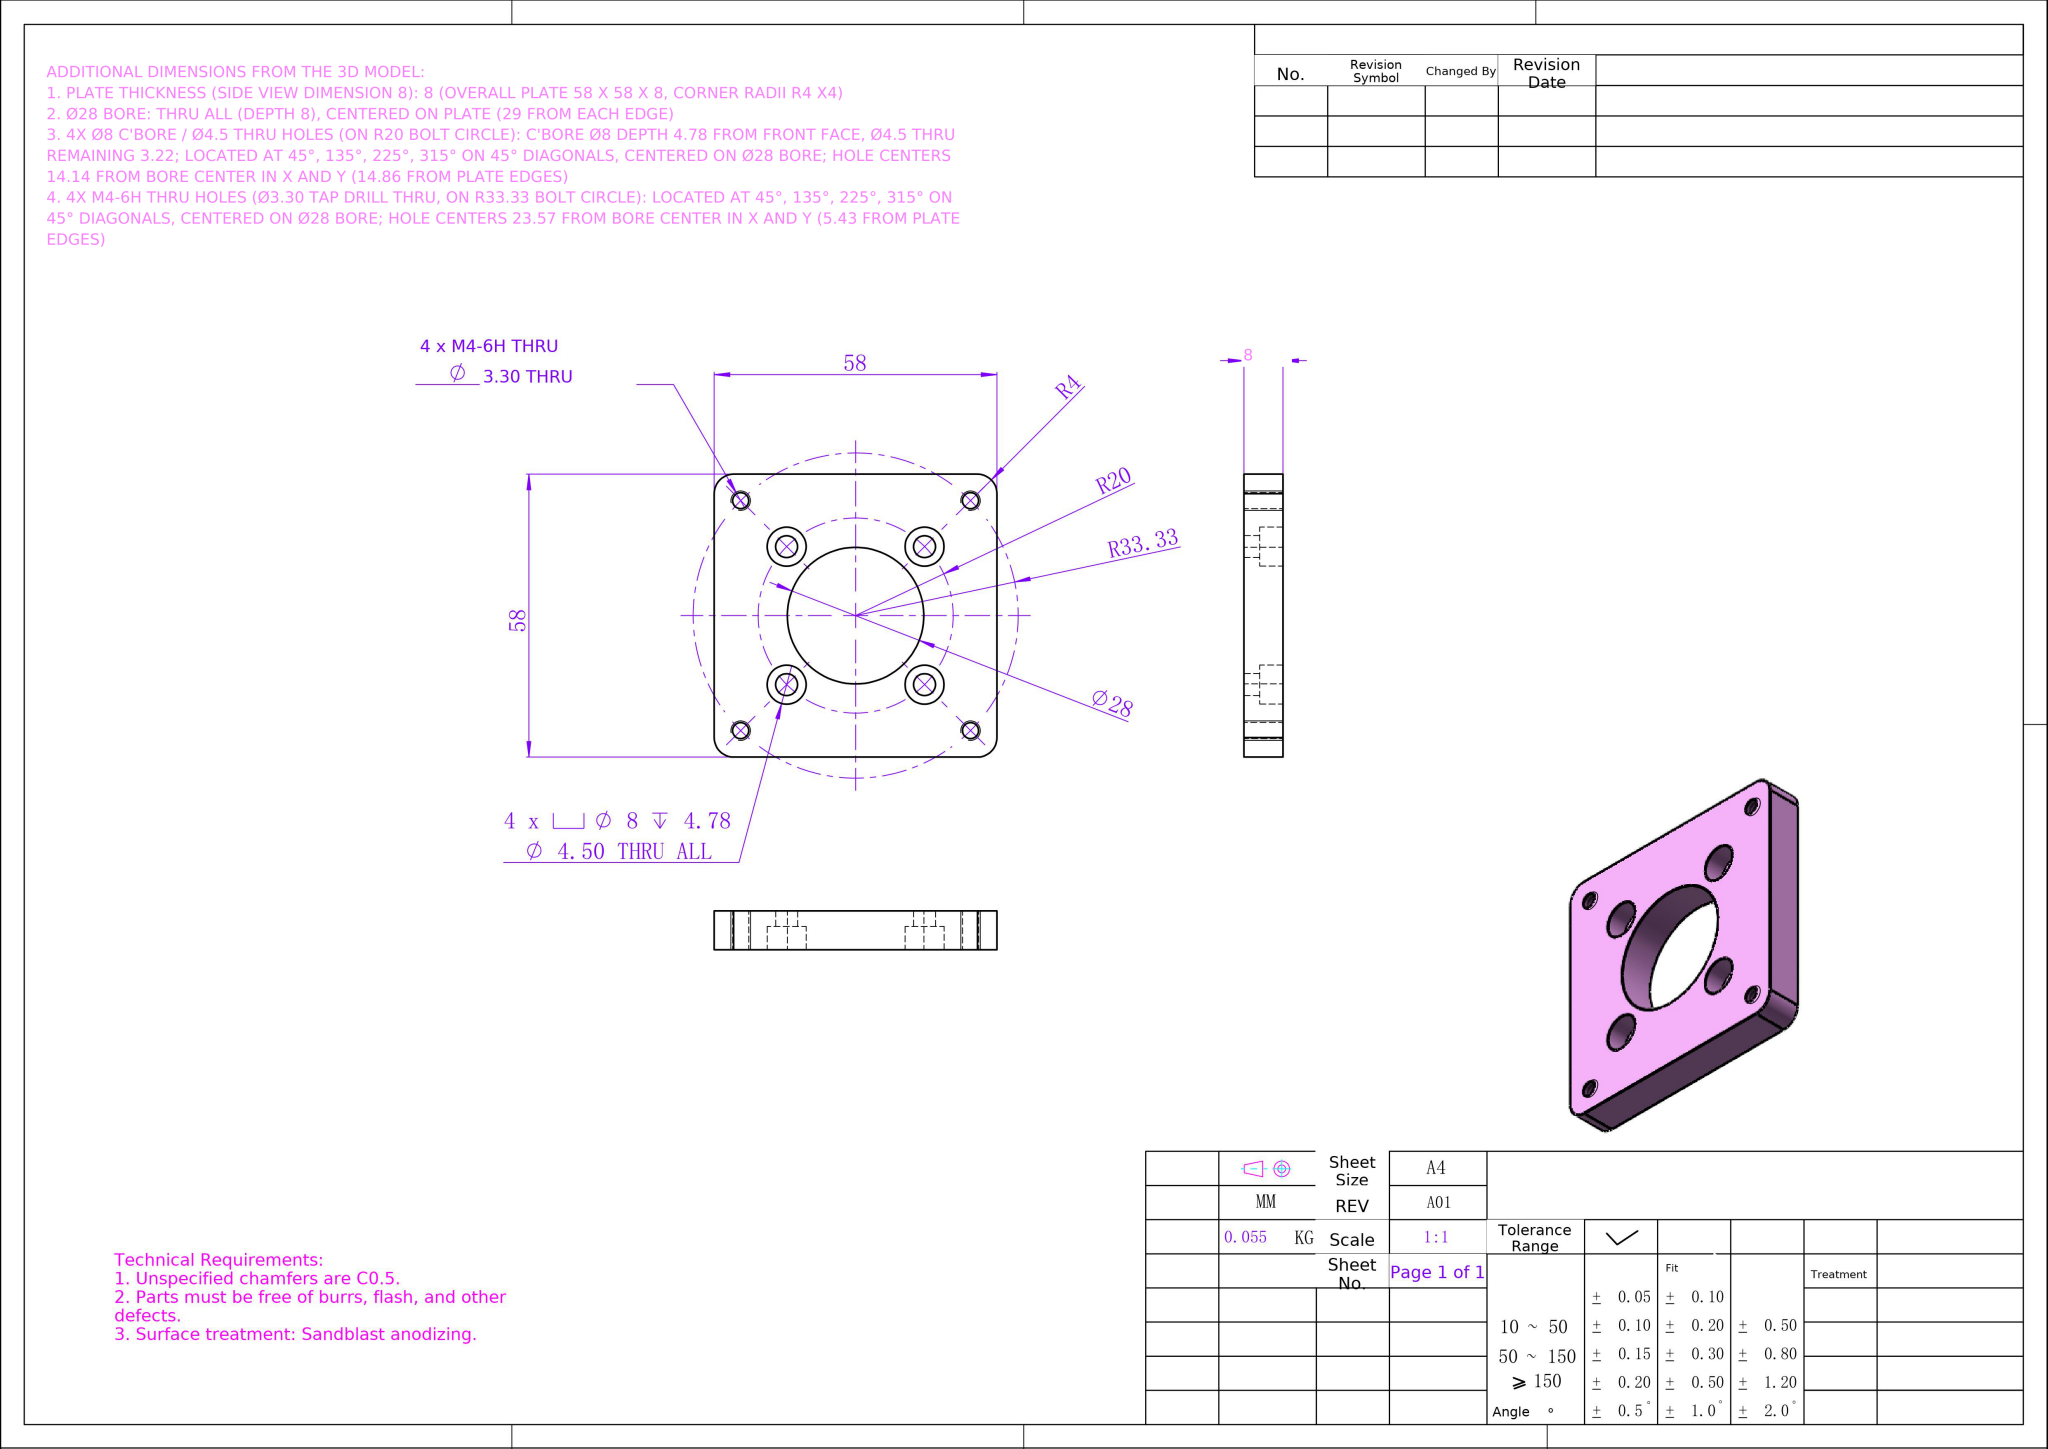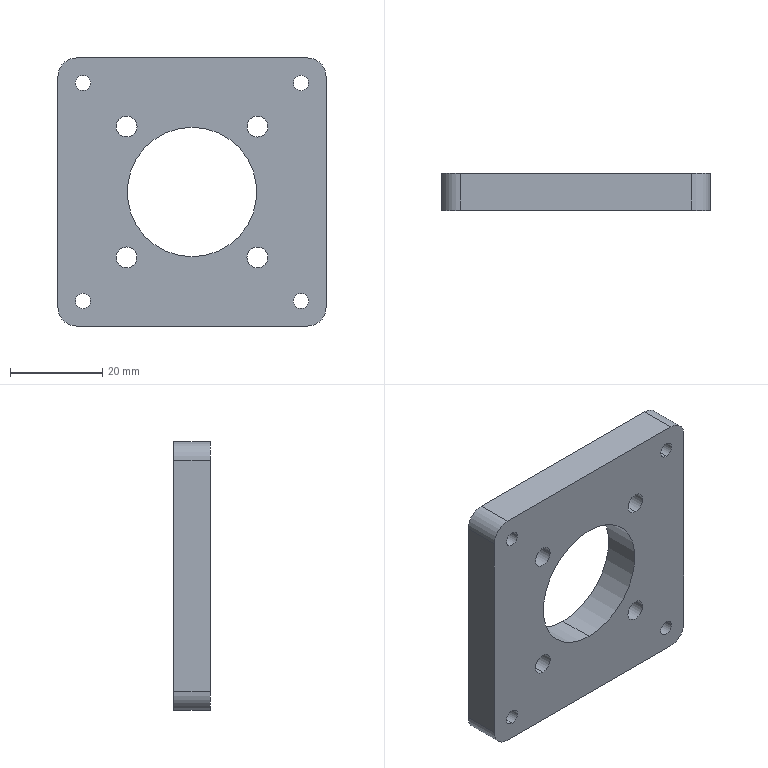Part | NX | mm | 1 solid | 40 faces | box 58 x 8 x 58 mm | volume 20437 mm3 | cylinder 30 | plane 10 | commonest cylinder face diameters 8 x12 3.3 x8 4.5 x8 28 x2